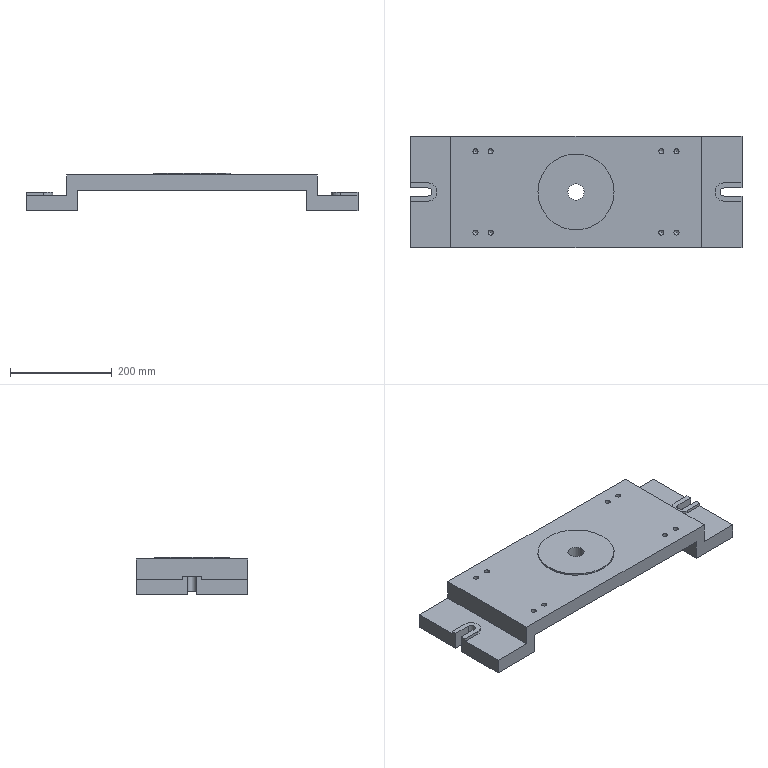Component | NX | FIXTURE_BODY | 1 solid | 57 faces | volume 4681377 mm3 | plane 31 | cylinder 16 | cone 10 | commonest cylinder face diameters 10 x8 16 x2 36 x2 6 x2 150 x1 32 x1